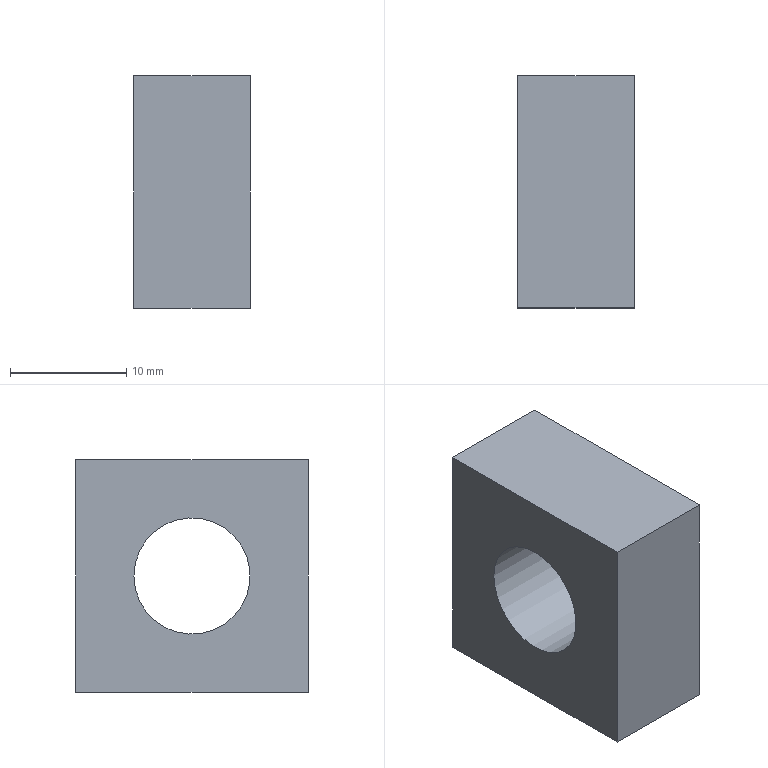Component | NX | BUSHING | 1 solid | 7 faces | box 10 x 20 x 20 mm | volume 3215 mm3 | plane 6 | cylinder 1 | commonest cylinder face diameters 10 x1
STEP:
#1=CARTESIAN_POINT('',(0.,0.,0.));
#2=DIRECTION('',(0.,0.,1.));
#3=DIRECTION('',(1.,0.,0.));
#4=AXIS2_PLACEMENT_3D('',#1,#2,#3);
#5=CARTESIAN_POINT('',(-49.,-10.,46.5));
#6=VERTEX_POINT('',#5);
#7=CARTESIAN_POINT('',(-49.,-10.,26.5));
#8=VERTEX_POINT('',#7);
#9=CARTESIAN_POINT('',(-49.,-10.,46.5));
#10=DIRECTION('',(0.,0.,-1.));
#11=VECTOR('',#10,1.);
#12=LINE('',#9,#11);
#13=CARTESIAN_POINT('',(-39.,-10.,46.5));
#14=DIRECTION('',(0.,1.,0.));
#15=DIRECTION('',(0.,0.,1.));
#16=AXIS2_PLACEMENT_3D('',#13,#14,#15);
#17=PLANE('',#16);
#18=CARTESIAN_POINT('',(0.,-10.));
#19=DIRECTION('',(-1.,0.));
#20=VECTOR('',#19,1.);
#21=LINE('',#18,#20);
#22=(GEOMETRIC_REPRESENTATION_CONTEXT(2)PARAMETRIC_REPRESENTATION_CONTEXT()REPRESENTATION_CONTEXT('',''));
#23=DEFINITIONAL_REPRESENTATION('',(#21),#22);
#24=PCURVE('',#17,#23);
#25=CARTESIAN_POINT('',(-49.,0.,36.5));
#26=DIRECTION('',(1.,0.,0.));
#27=DIRECTION('',(0.,0.,-1.));
#28=AXIS2_PLACEMENT_3D('',#25,#26,#27);
#29=PLANE('',#28);
#30=CARTESIAN_POINT('',(-10.,-10.));
#31=DIRECTION('',(1.,0.));
#32=VECTOR('',#31,1.);
#33=LINE('',#30,#32);
#34=(GEOMETRIC_REPRESENTATION_CONTEXT(2)PARAMETRIC_REPRESENTATION_CONTEXT()REPRESENTATION_CONTEXT('',''));
#35=DEFINITIONAL_REPRESENTATION('',(#33),#34);
#36=PCURVE('',#29,#35);
#37=SURFACE_CURVE('',#12,(#24,#36),.PCURVE_S1.);
#38=EDGE_CURVE('',#6,#8,#37,.T.);
#39=ORIENTED_EDGE('',*,*,#38,.T.);
#40=CARTESIAN_POINT('',(-39.,-10.,26.5));
#41=VERTEX_POINT('',#40);
#42=CARTESIAN_POINT('',(-39.,-10.,26.5));
#43=DIRECTION('',(-1.,0.,0.));
#44=VECTOR('',#43,1.);
#45=LINE('',#42,#44);
#46=CARTESIAN_POINT('',(-20.,0.));
#47=DIRECTION('',(0.,-1.));
#48=VECTOR('',#47,1.);
#49=LINE('',#46,#48);
#50=(GEOMETRIC_REPRESENTATION_CONTEXT(2)PARAMETRIC_REPRESENTATION_CONTEXT()REPRESENTATION_CONTEXT('',''));
#51=DEFINITIONAL_REPRESENTATION('',(#49),#50);
#52=PCURVE('',#17,#51);
#53=CARTESIAN_POINT('',(-39.,-10.,26.5));
#54=DIRECTION('',(0.,0.,1.));
#55=DIRECTION('',(1.,0.,0.));
#56=AXIS2_PLACEMENT_3D('',#53,#54,#55);
#57=PLANE('',#56);
#58=CARTESIAN_POINT('',(0.,0.));
#59=DIRECTION('',(-1.,0.));
#60=VECTOR('',#59,1.);
#61=LINE('',#58,#60);
#62=(GEOMETRIC_REPRESENTATION_CONTEXT(2)PARAMETRIC_REPRESENTATION_CONTEXT()REPRESENTATION_CONTEXT('',''));
#63=DEFINITIONAL_REPRESENTATION('',(#61),#62);
#64=PCURVE('',#57,#63);
#65=SURFACE_CURVE('',#45,(#52,#64),.PCURVE_S1.);
#66=EDGE_CURVE('',#41,#8,#65,.T.);
#67=ORIENTED_EDGE('',*,*,#66,.F.);
#68=CARTESIAN_POINT('',(-39.,-10.,46.5));
#69=VERTEX_POINT('',#68);
#70=CARTESIAN_POINT('',(-39.,-10.,46.5));
#71=DIRECTION('',(0.,0.,-1.));
#72=VECTOR('',#71,1.);
#73=LINE('',#70,#72);
#74=CARTESIAN_POINT('',(0.,0.));
#75=DIRECTION('',(-1.,0.));
#76=VECTOR('',#75,1.);
#77=LINE('',#74,#76);
#78=(GEOMETRIC_REPRESENTATION_CONTEXT(2)PARAMETRIC_REPRESENTATION_CONTEXT()REPRESENTATION_CONTEXT('',''));
#79=DEFINITIONAL_REPRESENTATION('',(#77),#78);
#80=PCURVE('',#17,#79);
#81=CARTESIAN_POINT('',(-39.,0.,36.5));
#82=DIRECTION('',(1.,0.,0.));
#83=DIRECTION('',(0.,0.,-1.));
#84=AXIS2_PLACEMENT_3D('',#81,#82,#83);
#85=PLANE('',#84);
#86=CARTESIAN_POINT('',(-10.,-10.));
#87=DIRECTION('',(1.,0.));
#88=VECTOR('',#87,1.);
#89=LINE('',#86,#88);
#90=(GEOMETRIC_REPRESENTATION_CONTEXT(2)PARAMETRIC_REPRESENTATION_CONTEXT()REPRESENTATION_CONTEXT('',''));
#91=DEFINITIONAL_REPRESENTATION('',(#89),#90);
#92=PCURVE('',#85,#91);
#93=SURFACE_CURVE('',#73,(#80,#92),.PCURVE_S1.);
#94=EDGE_CURVE('',#69,#41,#93,.T.);
#95=ORIENTED_EDGE('',*,*,#94,.F.);
#96=CARTESIAN_POINT('',(-39.,-10.,46.5));
#97=DIRECTION('',(-1.,0.,0.));
#98=VECTOR('',#97,1.);
#99=LINE('',#96,#98);
#100=CARTESIAN_POINT('',(0.,0.));
#101=DIRECTION('',(0.,-1.));
#102=VECTOR('',#101,1.);
#103=LINE('',#100,#102);
#104=(GEOMETRIC_REPRESENTATION_CONTEXT(2)PARAMETRIC_REPRESENTATION_CONTEXT()REPRESENTATION_CONTEXT('',''));
#105=DEFINITIONAL_REPRESENTATION('',(#103),#104);
#106=PCURVE('',#17,#105);
#107=CARTESIAN_POINT('',(-39.,10.,46.5));
#108=DIRECTION('',(0.,0.,-1.));
#109=DIRECTION('',(-1.,0.,0.));
#110=AXIS2_PLACEMENT_3D('',#107,#108,#109);
#111=PLANE('',#110);
#112=CARTESIAN_POINT('',(0.,-20.));
#113=DIRECTION('',(1.,0.));
#114=VECTOR('',#113,1.);
#115=LINE('',#112,#114);
#116=(GEOMETRIC_REPRESENTATION_CONTEXT(2)PARAMETRIC_REPRESENTATION_CONTEXT()REPRESENTATION_CONTEXT('',''));
#117=DEFINITIONAL_REPRESENTATION('',(#115),#116);
#118=PCURVE('',#111,#117);
#119=SURFACE_CURVE('',#99,(#106,#118),.PCURVE_S1.);
#120=EDGE_CURVE('',#69,#6,#119,.T.);
#121=ORIENTED_EDGE('',*,*,#120,.T.);
#122=EDGE_LOOP('',(#39,#67,#95,#121));
#123=FACE_BOUND('',#122,.T.);
#124=ADVANCED_FACE('',(#123),#17,.F.);
#125=CARTESIAN_POINT('',(-49.,10.,26.5));
#126=VERTEX_POINT('',#125);
#127=CARTESIAN_POINT('',(-49.,-10.,26.5));
#128=DIRECTION('',(0.,1.,0.));
#129=VECTOR('',#128,1.);
#130=LINE('',#127,#129);
#131=CARTESIAN_POINT('',(-10.,0.));
#132=DIRECTION('',(0.,1.));
#133=VECTOR('',#132,1.);
#134=LINE('',#131,#133);
#135=(GEOMETRIC_REPRESENTATION_CONTEXT(2)PARAMETRIC_REPRESENTATION_CONTEXT()REPRESENTATION_CONTEXT('',''));
#136=DEFINITIONAL_REPRESENTATION('',(#134),#135);
#137=PCURVE('',#57,#136);
#138=CARTESIAN_POINT('',(10.,-10.));
#139=DIRECTION('',(0.,1.));
#140=VECTOR('',#139,1.);
#141=LINE('',#138,#140);
#142=(GEOMETRIC_REPRESENTATION_CONTEXT(2)PARAMETRIC_REPRESENTATION_CONTEXT()REPRESENTATION_CONTEXT('',''));
#143=DEFINITIONAL_REPRESENTATION('',(#141),#142);
#144=PCURVE('',#29,#143);
#145=SURFACE_CURVE('',#130,(#137,#144),.PCURVE_S1.);
#146=EDGE_CURVE('',#8,#126,#145,.T.);
#147=ORIENTED_EDGE('',*,*,#146,.T.);
#148=CARTESIAN_POINT('',(-39.,10.,26.5));
#149=VERTEX_POINT('',#148);
#150=CARTESIAN_POINT('',(-39.,10.,26.5));
#151=DIRECTION('',(-1.,0.,0.));
#152=VECTOR('',#151,1.);
#153=LINE('',#150,#152);
#154=CARTESIAN_POINT('',(0.,20.));
#155=DIRECTION('',(-1.,0.));
#156=VECTOR('',#155,1.);
#157=LINE('',#154,#156);
#158=(GEOMETRIC_REPRESENTATION_CONTEXT(2)PARAMETRIC_REPRESENTATION_CONTEXT()REPRESENTATION_CONTEXT('',''));
#159=DEFINITIONAL_REPRESENTATION('',(#157),#158);
#160=PCURVE('',#57,#159);
#161=CARTESIAN_POINT('',(-39.,10.,26.5));
#162=DIRECTION('',(0.,-1.,0.));
#163=DIRECTION('',(0.,0.,-1.));
#164=AXIS2_PLACEMENT_3D('',#161,#162,#163);
#165=PLANE('',#164);
#166=CARTESIAN_POINT('',(0.,0.));
#167=DIRECTION('',(0.,-1.));
#168=VECTOR('',#167,1.);
#169=LINE('',#166,#168);
#170=(GEOMETRIC_REPRESENTATION_CONTEXT(2)PARAMETRIC_REPRESENTATION_CONTEXT()REPRESENTATION_CONTEXT('',''));
#171=DEFINITIONAL_REPRESENTATION('',(#169),#170);
#172=PCURVE('',#165,#171);
#173=SURFACE_CURVE('',#153,(#160,#172),.PCURVE_S1.);
#174=EDGE_CURVE('',#149,#126,#173,.T.);
#175=ORIENTED_EDGE('',*,*,#174,.F.);
#176=CARTESIAN_POINT('',(-39.,-10.,26.5));
#177=DIRECTION('',(0.,1.,0.));
#178=VECTOR('',#177,1.);
#179=LINE('',#176,#178);
#180=CARTESIAN_POINT('',(0.,0.));
#181=DIRECTION('',(0.,1.));
#182=VECTOR('',#181,1.);
#183=LINE('',#180,#182);
#184=(GEOMETRIC_REPRESENTATION_CONTEXT(2)PARAMETRIC_REPRESENTATION_CONTEXT()REPRESENTATION_CONTEXT('',''));
#185=DEFINITIONAL_REPRESENTATION('',(#183),#184);
#186=PCURVE('',#57,#185);
#187=CARTESIAN_POINT('',(10.,-10.));
#188=DIRECTION('',(0.,1.));
#189=VECTOR('',#188,1.);
#190=LINE('',#187,#189);
#191=(GEOMETRIC_REPRESENTATION_CONTEXT(2)PARAMETRIC_REPRESENTATION_CONTEXT()REPRESENTATION_CONTEXT('',''));
#192=DEFINITIONAL_REPRESENTATION('',(#190),#191);
#193=PCURVE('',#85,#192);
#194=SURFACE_CURVE('',#179,(#186,#193),.PCURVE_S1.);
#195=EDGE_CURVE('',#41,#149,#194,.T.);
#196=ORIENTED_EDGE('',*,*,#195,.F.);
#197=ORIENTED_EDGE('',*,*,#66,.T.);
#198=EDGE_LOOP('',(#147,#175,#196,#197));
#199=FACE_BOUND('',#198,.T.);
#200=ADVANCED_FACE('',(#199),#57,.F.);
#201=CARTESIAN_POINT('',(-49.,10.,46.5));
#202=VERTEX_POINT('',#201);
#203=CARTESIAN_POINT('',(-49.,10.,26.5));
#204=DIRECTION('',(0.,0.,1.));
#205=VECTOR('',#204,1.);
#206=LINE('',#203,#205);
#207=CARTESIAN_POINT('',(0.,-10.));
#208=DIRECTION('',(-1.,0.));
#209=VECTOR('',#208,1.);
#210=LINE('',#207,#209);
#211=(GEOMETRIC_REPRESENTATION_CONTEXT(2)PARAMETRIC_REPRESENTATION_CONTEXT()REPRESENTATION_CONTEXT('',''));
#212=DEFINITIONAL_REPRESENTATION('',(#210),#211);
#213=PCURVE('',#165,#212);
#214=CARTESIAN_POINT('',(10.,10.));
#215=DIRECTION('',(-1.,0.));
#216=VECTOR('',#215,1.);
#217=LINE('',#214,#216);
#218=(GEOMETRIC_REPRESENTATION_CONTEXT(2)PARAMETRIC_REPRESENTATION_CONTEXT()REPRESENTATION_CONTEXT('',''));
#219=DEFINITIONAL_REPRESENTATION('',(#217),#218);
#220=PCURVE('',#29,#219);
#221=SURFACE_CURVE('',#206,(#213,#220),.PCURVE_S1.);
#222=EDGE_CURVE('',#126,#202,#221,.T.);
#223=ORIENTED_EDGE('',*,*,#222,.T.);
#224=CARTESIAN_POINT('',(-39.,10.,46.5));
#225=VERTEX_POINT('',#224);
#226=CARTESIAN_POINT('',(-39.,10.,46.5));
#227=DIRECTION('',(-1.,0.,0.));
#228=VECTOR('',#227,1.);
#229=LINE('',#226,#228);
#230=CARTESIAN_POINT('',(-20.,0.));
#231=DIRECTION('',(0.,-1.));
#232=VECTOR('',#231,1.);
#233=LINE('',#230,#232);
#234=(GEOMETRIC_REPRESENTATION_CONTEXT(2)PARAMETRIC_REPRESENTATION_CONTEXT()REPRESENTATION_CONTEXT('',''));
#235=DEFINITIONAL_REPRESENTATION('',(#233),#234);
#236=PCURVE('',#165,#235);
#237=CARTESIAN_POINT('',(0.,0.));
#238=DIRECTION('',(1.,0.));
#239=VECTOR('',#238,1.);
#240=LINE('',#237,#239);
#241=(GEOMETRIC_REPRESENTATION_CONTEXT(2)PARAMETRIC_REPRESENTATION_CONTEXT()REPRESENTATION_CONTEXT('',''));
#242=DEFINITIONAL_REPRESENTATION('',(#240),#241);
#243=PCURVE('',#111,#242);
#244=SURFACE_CURVE('',#229,(#236,#243),.PCURVE_S1.);
#245=EDGE_CURVE('',#225,#202,#244,.T.);
#246=ORIENTED_EDGE('',*,*,#245,.F.);
#247=CARTESIAN_POINT('',(-39.,10.,26.5));
#248=DIRECTION('',(0.,0.,1.));
#249=VECTOR('',#248,1.);
#250=LINE('',#247,#249);
#251=CARTESIAN_POINT('',(0.,0.));
#252=DIRECTION('',(-1.,0.));
#253=VECTOR('',#252,1.);
#254=LINE('',#251,#253);
#255=(GEOMETRIC_REPRESENTATION_CONTEXT(2)PARAMETRIC_REPRESENTATION_CONTEXT()REPRESENTATION_CONTEXT('',''));
#256=DEFINITIONAL_REPRESENTATION('',(#254),#255);
#257=PCURVE('',#165,#256);
#258=CARTESIAN_POINT('',(10.,10.));
#259=DIRECTION('',(-1.,0.));
#260=VECTOR('',#259,1.);
#261=LINE('',#258,#260);
#262=(GEOMETRIC_REPRESENTATION_CONTEXT(2)PARAMETRIC_REPRESENTATION_CONTEXT()REPRESENTATION_CONTEXT('',''));
#263=DEFINITIONAL_REPRESENTATION('',(#261),#262);
#264=PCURVE('',#85,#263);
#265=SURFACE_CURVE('',#250,(#257,#264),.PCURVE_S1.);
#266=EDGE_CURVE('',#149,#225,#265,.T.);
#267=ORIENTED_EDGE('',*,*,#266,.F.);
#268=ORIENTED_EDGE('',*,*,#174,.T.);
#269=EDGE_LOOP('',(#223,#246,#267,#268));
#270=FACE_BOUND('',#269,.T.);
#271=ADVANCED_FACE('',(#270),#165,.F.);
#272=CARTESIAN_POINT('',(-49.,10.,46.5));
#273=DIRECTION('',(0.,-1.,0.));
#274=VECTOR('',#273,1.);
#275=LINE('',#272,#274);
#276=CARTESIAN_POINT('',(10.,0.));
#277=DIRECTION('',(0.,-1.));
#278=VECTOR('',#277,1.);
#279=LINE('',#276,#278);
#280=(GEOMETRIC_REPRESENTATION_CONTEXT(2)PARAMETRIC_REPRESENTATION_CONTEXT()REPRESENTATION_CONTEXT('',''));
#281=DEFINITIONAL_REPRESENTATION('',(#279),#280);
#282=PCURVE('',#111,#281);
#283=CARTESIAN_POINT('',(-10.,10.));
#284=DIRECTION('',(0.,-1.));
#285=VECTOR('',#284,1.);
#286=LINE('',#283,#285);
#287=(GEOMETRIC_REPRESENTATION_CONTEXT(2)PARAMETRIC_REPRESENTATION_CONTEXT()REPRESENTATION_CONTEXT('',''));
#288=DEFINITIONAL_REPRESENTATION('',(#286),#287);
#289=PCURVE('',#29,#288);
#290=SURFACE_CURVE('',#275,(#282,#289),.PCURVE_S1.);
#291=EDGE_CURVE('',#202,#6,#290,.T.);
#292=ORIENTED_EDGE('',*,*,#291,.T.);
#293=ORIENTED_EDGE('',*,*,#120,.F.);
#294=CARTESIAN_POINT('',(-39.,10.,46.5));
#295=DIRECTION('',(0.,-1.,0.));
#296=VECTOR('',#295,1.);
#297=LINE('',#294,#296);
#298=CARTESIAN_POINT('',(0.,0.));
#299=DIRECTION('',(0.,-1.));
#300=VECTOR('',#299,1.);
#301=LINE('',#298,#300);
#302=(GEOMETRIC_REPRESENTATION_CONTEXT(2)PARAMETRIC_REPRESENTATION_CONTEXT()REPRESENTATION_CONTEXT('',''));
#303=DEFINITIONAL_REPRESENTATION('',(#301),#302);
#304=PCURVE('',#111,#303);
#305=CARTESIAN_POINT('',(-10.,10.));
#306=DIRECTION('',(0.,-1.));
#307=VECTOR('',#306,1.);
#308=LINE('',#305,#307);
#309=(GEOMETRIC_REPRESENTATION_CONTEXT(2)PARAMETRIC_REPRESENTATION_CONTEXT()REPRESENTATION_CONTEXT('',''));
#310=DEFINITIONAL_REPRESENTATION('',(#308),#309);
#311=PCURVE('',#85,#310);
#312=SURFACE_CURVE('',#297,(#304,#311),.PCURVE_S1.);
#313=EDGE_CURVE('',#225,#69,#312,.T.);
#314=ORIENTED_EDGE('',*,*,#313,.F.);
#315=ORIENTED_EDGE('',*,*,#245,.T.);
#316=EDGE_LOOP('',(#292,#293,#314,#315));
#317=FACE_BOUND('',#316,.T.);
#318=ADVANCED_FACE('',(#317),#111,.F.);
#319=CARTESIAN_POINT('',(-39.,5.,36.5));
#320=VERTEX_POINT('',#319);
#321=CARTESIAN_POINT('',(-39.,0.,36.5));
#322=DIRECTION('',(1.,0.,0.));
#323=DIRECTION('',(0.,1.,0.));
#324=AXIS2_PLACEMENT_3D('',#321,#322,#323);
#325=CIRCLE('',#324,5.);
#326=CARTESIAN_POINT('',(-39.,0.,36.5));
#327=DIRECTION('',(-1.,0.,0.));
#328=DIRECTION('',(0.,0.,1.));
#329=AXIS2_PLACEMENT_3D('',#326,#327,#328);
#330=CYLINDRICAL_SURFACE('',#329,5.);
#331=CARTESIAN_POINT('',(7.854,0.));
#332=DIRECTION('',(-1.,0.));
#333=VECTOR('',#332,1.);
#334=LINE('',#331,#333);
#335=(GEOMETRIC_REPRESENTATION_CONTEXT(2)PARAMETRIC_REPRESENTATION_CONTEXT()REPRESENTATION_CONTEXT('',''));
#336=DEFINITIONAL_REPRESENTATION('',(#334),#335);
#337=PCURVE('',#330,#336);
#338=CARTESIAN_POINT('',(0.,0.));
#339=DIRECTION('',(0.,1.));
#340=AXIS2_PLACEMENT_2D('',#338,#339);
#341=CIRCLE('',#340,5.);
#342=(GEOMETRIC_REPRESENTATION_CONTEXT(2)PARAMETRIC_REPRESENTATION_CONTEXT()REPRESENTATION_CONTEXT('',''));
#343=DEFINITIONAL_REPRESENTATION('',(#341),#342);
#344=PCURVE('',#85,#343);
#345=SURFACE_CURVE('',#325,(#337,#344),.PCURVE_S1.);
#346=EDGE_CURVE('',#320,#320,#345,.T.);
#347=ORIENTED_EDGE('',*,*,#346,.F.);
#348=CARTESIAN_POINT('',(-49.,5.,36.5));
#349=VERTEX_POINT('',#348);
#350=CARTESIAN_POINT('',(-39.,5.,36.5));
#351=CARTESIAN_POINT('',(-49.,5.,36.5));
#352=B_SPLINE_CURVE_WITH_KNOTS('',1,(#350,#351),.UNSPECIFIED.,.F.,.F.,(2,2),(0.,10.),.PIECEWISE_BEZIER_KNOTS.);
#353=CARTESIAN_POINT('',(7.854,0.));
#354=DIRECTION('',(0.,1.));
#355=VECTOR('',#354,1.);
#356=LINE('',#353,#355);
#357=(GEOMETRIC_REPRESENTATION_CONTEXT(2)PARAMETRIC_REPRESENTATION_CONTEXT()REPRESENTATION_CONTEXT('',''));
#358=DEFINITIONAL_REPRESENTATION('',(#356),#357);
#359=PCURVE('',#330,#358);
#360=CARTESIAN_POINT('',(1.571,0.));
#361=DIRECTION('',(0.,1.));
#362=VECTOR('',#361,1.);
#363=LINE('',#360,#362);
#364=(GEOMETRIC_REPRESENTATION_CONTEXT(2)PARAMETRIC_REPRESENTATION_CONTEXT()REPRESENTATION_CONTEXT('',''));
#365=DEFINITIONAL_REPRESENTATION('',(#363),#364);
#366=PCURVE('',#330,#365);
#367=SEAM_CURVE('',#352,(#359,#366),.PCURVE_S1.);
#368=EDGE_CURVE('',#320,#349,#367,.T.);
#369=ORIENTED_EDGE('',*,*,#368,.T.);
#370=CARTESIAN_POINT('',(-49.,0.,36.5));
#371=DIRECTION('',(1.,0.,0.));
#372=DIRECTION('',(0.,1.,0.));
#373=AXIS2_PLACEMENT_3D('',#370,#371,#372);
#374=CIRCLE('',#373,5.);
#375=CARTESIAN_POINT('',(7.854,10.));
#376=DIRECTION('',(-1.,0.));
#377=VECTOR('',#376,1.);
#378=LINE('',#375,#377);
#379=(GEOMETRIC_REPRESENTATION_CONTEXT(2)PARAMETRIC_REPRESENTATION_CONTEXT()REPRESENTATION_CONTEXT('',''));
#380=DEFINITIONAL_REPRESENTATION('',(#378),#379);
#381=PCURVE('',#330,#380);
#382=CARTESIAN_POINT('',(0.,0.));
#383=DIRECTION('',(0.,1.));
#384=AXIS2_PLACEMENT_2D('',#382,#383);
#385=CIRCLE('',#384,5.);
#386=(GEOMETRIC_REPRESENTATION_CONTEXT(2)PARAMETRIC_REPRESENTATION_CONTEXT()REPRESENTATION_CONTEXT('',''));
#387=DEFINITIONAL_REPRESENTATION('',(#385),#386);
#388=PCURVE('',#29,#387);
#389=SURFACE_CURVE('',#374,(#381,#388),.PCURVE_S1.);
#390=EDGE_CURVE('',#349,#349,#389,.T.);
#391=ORIENTED_EDGE('',*,*,#390,.T.);
#392=ORIENTED_EDGE('',*,*,#368,.F.);
#393=EDGE_LOOP('',(#347,#369,#391,#392));
#394=FACE_BOUND('',#393,.F.);
#395=ADVANCED_FACE('',(#394),#330,.F.);
#396=ORIENTED_EDGE('',*,*,#94,.T.);
#397=ORIENTED_EDGE('',*,*,#195,.T.);
#398=ORIENTED_EDGE('',*,*,#266,.T.);
#399=ORIENTED_EDGE('',*,*,#313,.T.);
#400=EDGE_LOOP('',(#396,#397,#398,#399));
#401=FACE_BOUND('',#400,.T.);
#402=ORIENTED_EDGE('',*,*,#346,.F.);
#403=EDGE_LOOP('',(#402));
#404=FACE_BOUND('',#403,.T.);
#405=ADVANCED_FACE('',(#401,#404),#85,.T.);
#406=ORIENTED_EDGE('',*,*,#38,.F.);
#407=ORIENTED_EDGE('',*,*,#291,.F.);
#408=ORIENTED_EDGE('',*,*,#222,.F.);
#409=ORIENTED_EDGE('',*,*,#146,.F.);
#410=EDGE_LOOP('',(#406,#407,#408,#409));
#411=FACE_BOUND('',#410,.T.);
#412=ORIENTED_EDGE('',*,*,#390,.T.);
#413=EDGE_LOOP('',(#412));
#414=FACE_BOUND('',#413,.T.);
#415=ADVANCED_FACE('',(#411,#414),#29,.F.);
#416=CLOSED_SHELL('',(#124,#200,#271,#318,#395,#405,#415));
#417=MANIFOLD_SOLID_BREP('',#416);
#418=(LENGTH_UNIT()NAMED_UNIT(*)SI_UNIT(.MILLI.,.METRE.));
#419=UNCERTAINTY_MEASURE_WITH_UNIT(LENGTH_MEASURE(0.000002),#418,'','');
#420=(NAMED_UNIT(*)PLANE_ANGLE_UNIT()SI_UNIT($,.RADIAN.));
#421=(NAMED_UNIT(*)SI_UNIT($,.STERADIAN.)SOLID_ANGLE_UNIT());
#422=(GEOMETRIC_REPRESENTATION_CONTEXT(3)GLOBAL_UNCERTAINTY_ASSIGNED_CONTEXT((#419))GLOBAL_UNIT_ASSIGNED_CONTEXT((#418,#420,#421))REPRESENTATION_CONTEXT('',''));
#423=ADVANCED_BREP_SHAPE_REPRESENTATION('',(#4,#417),#422);